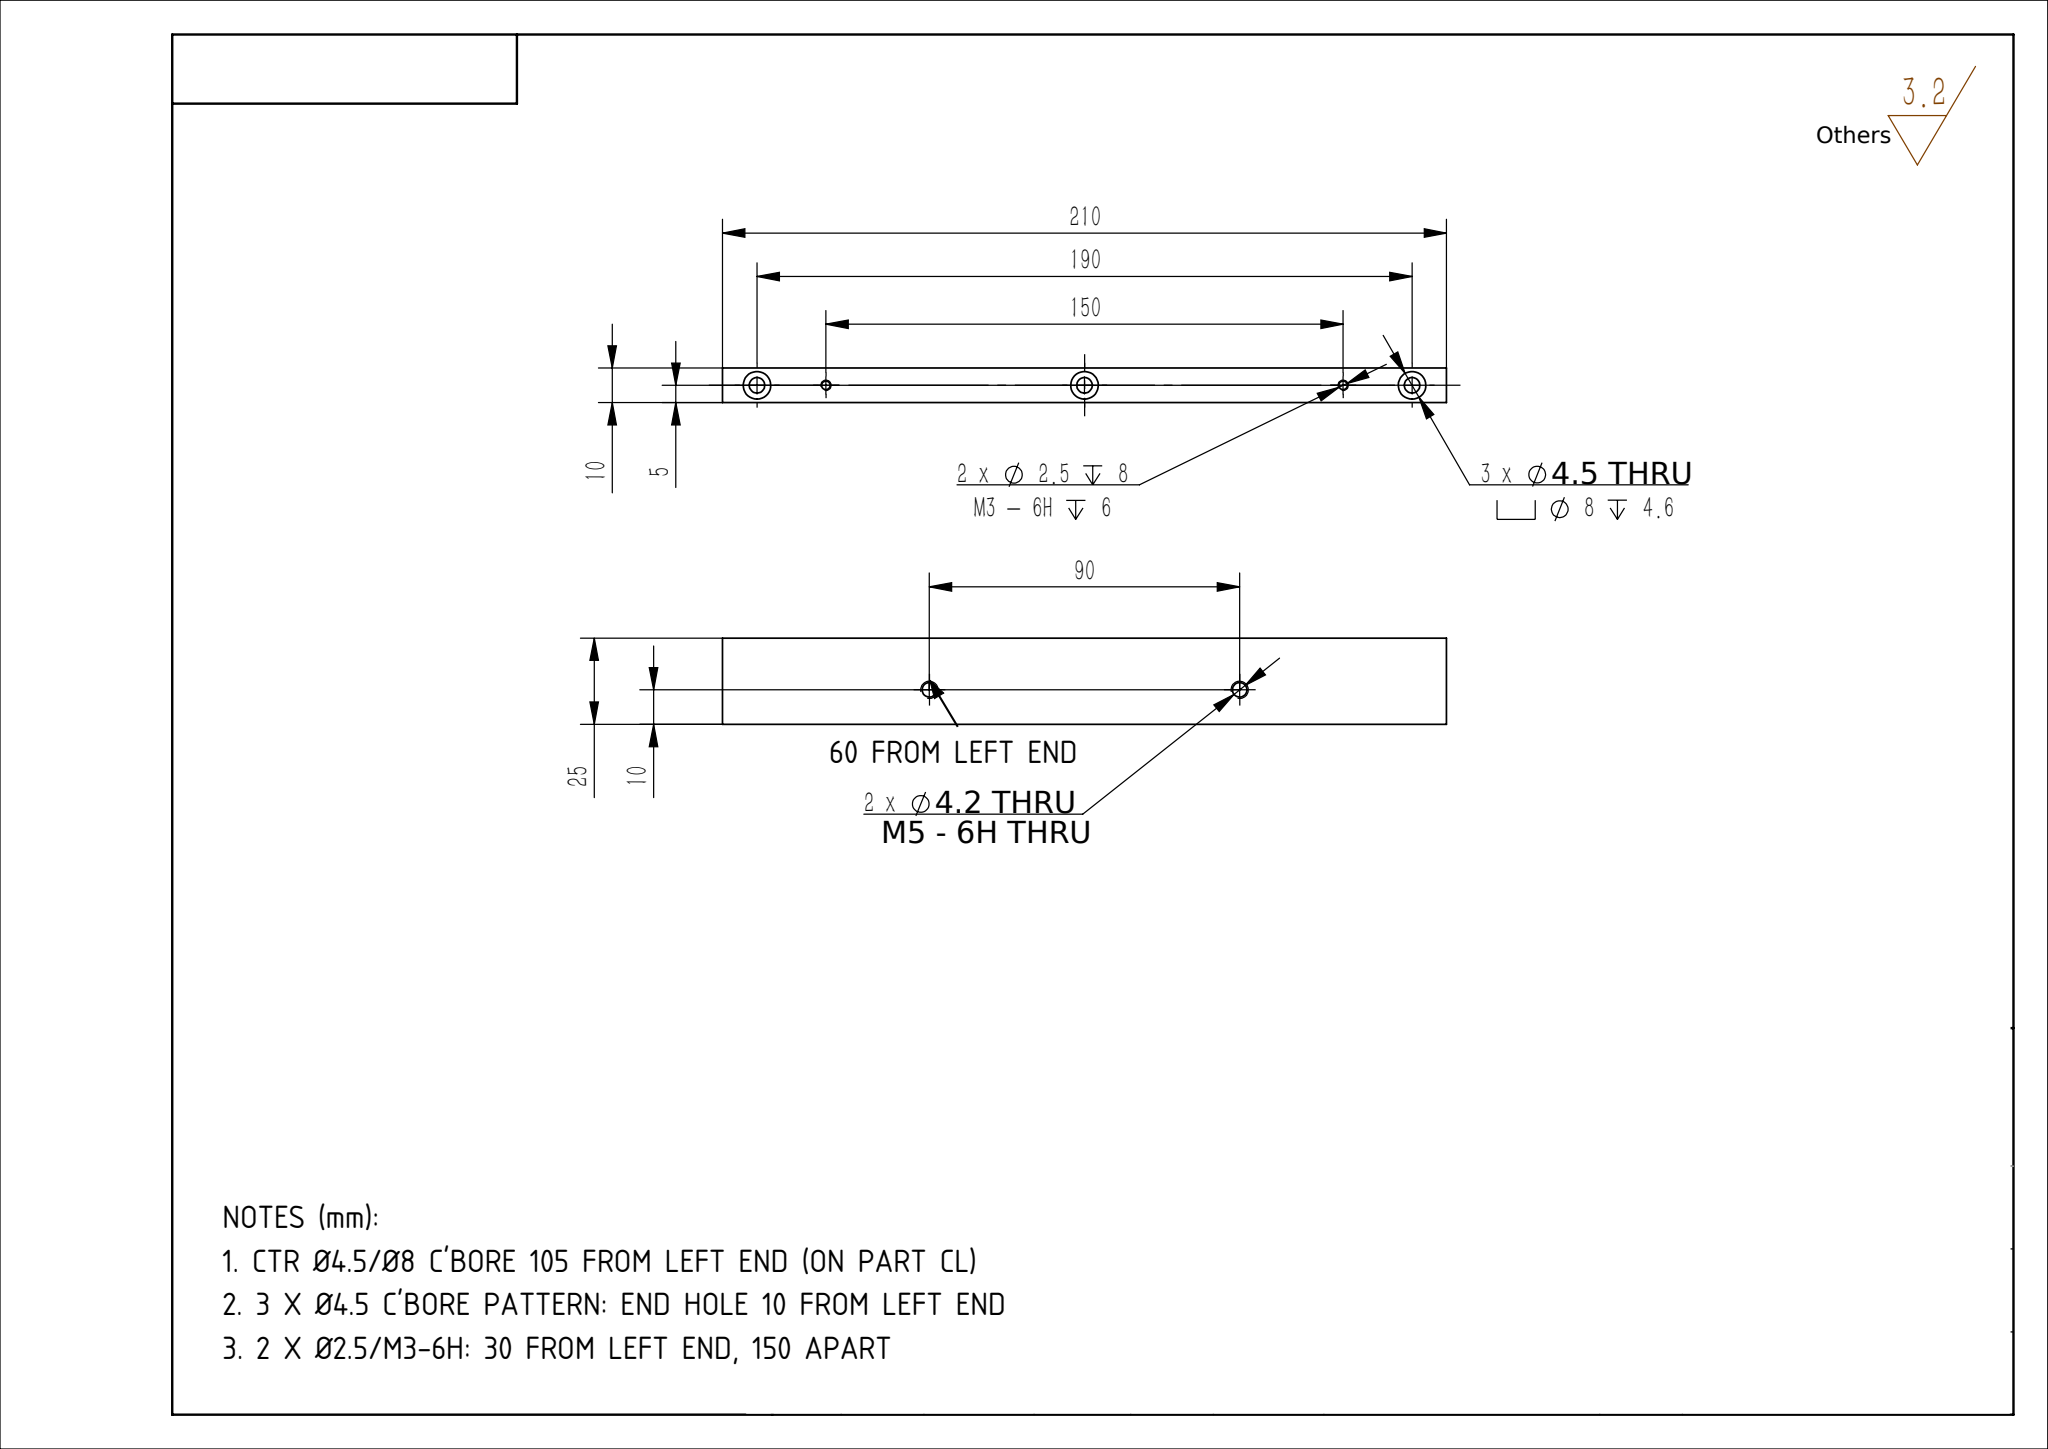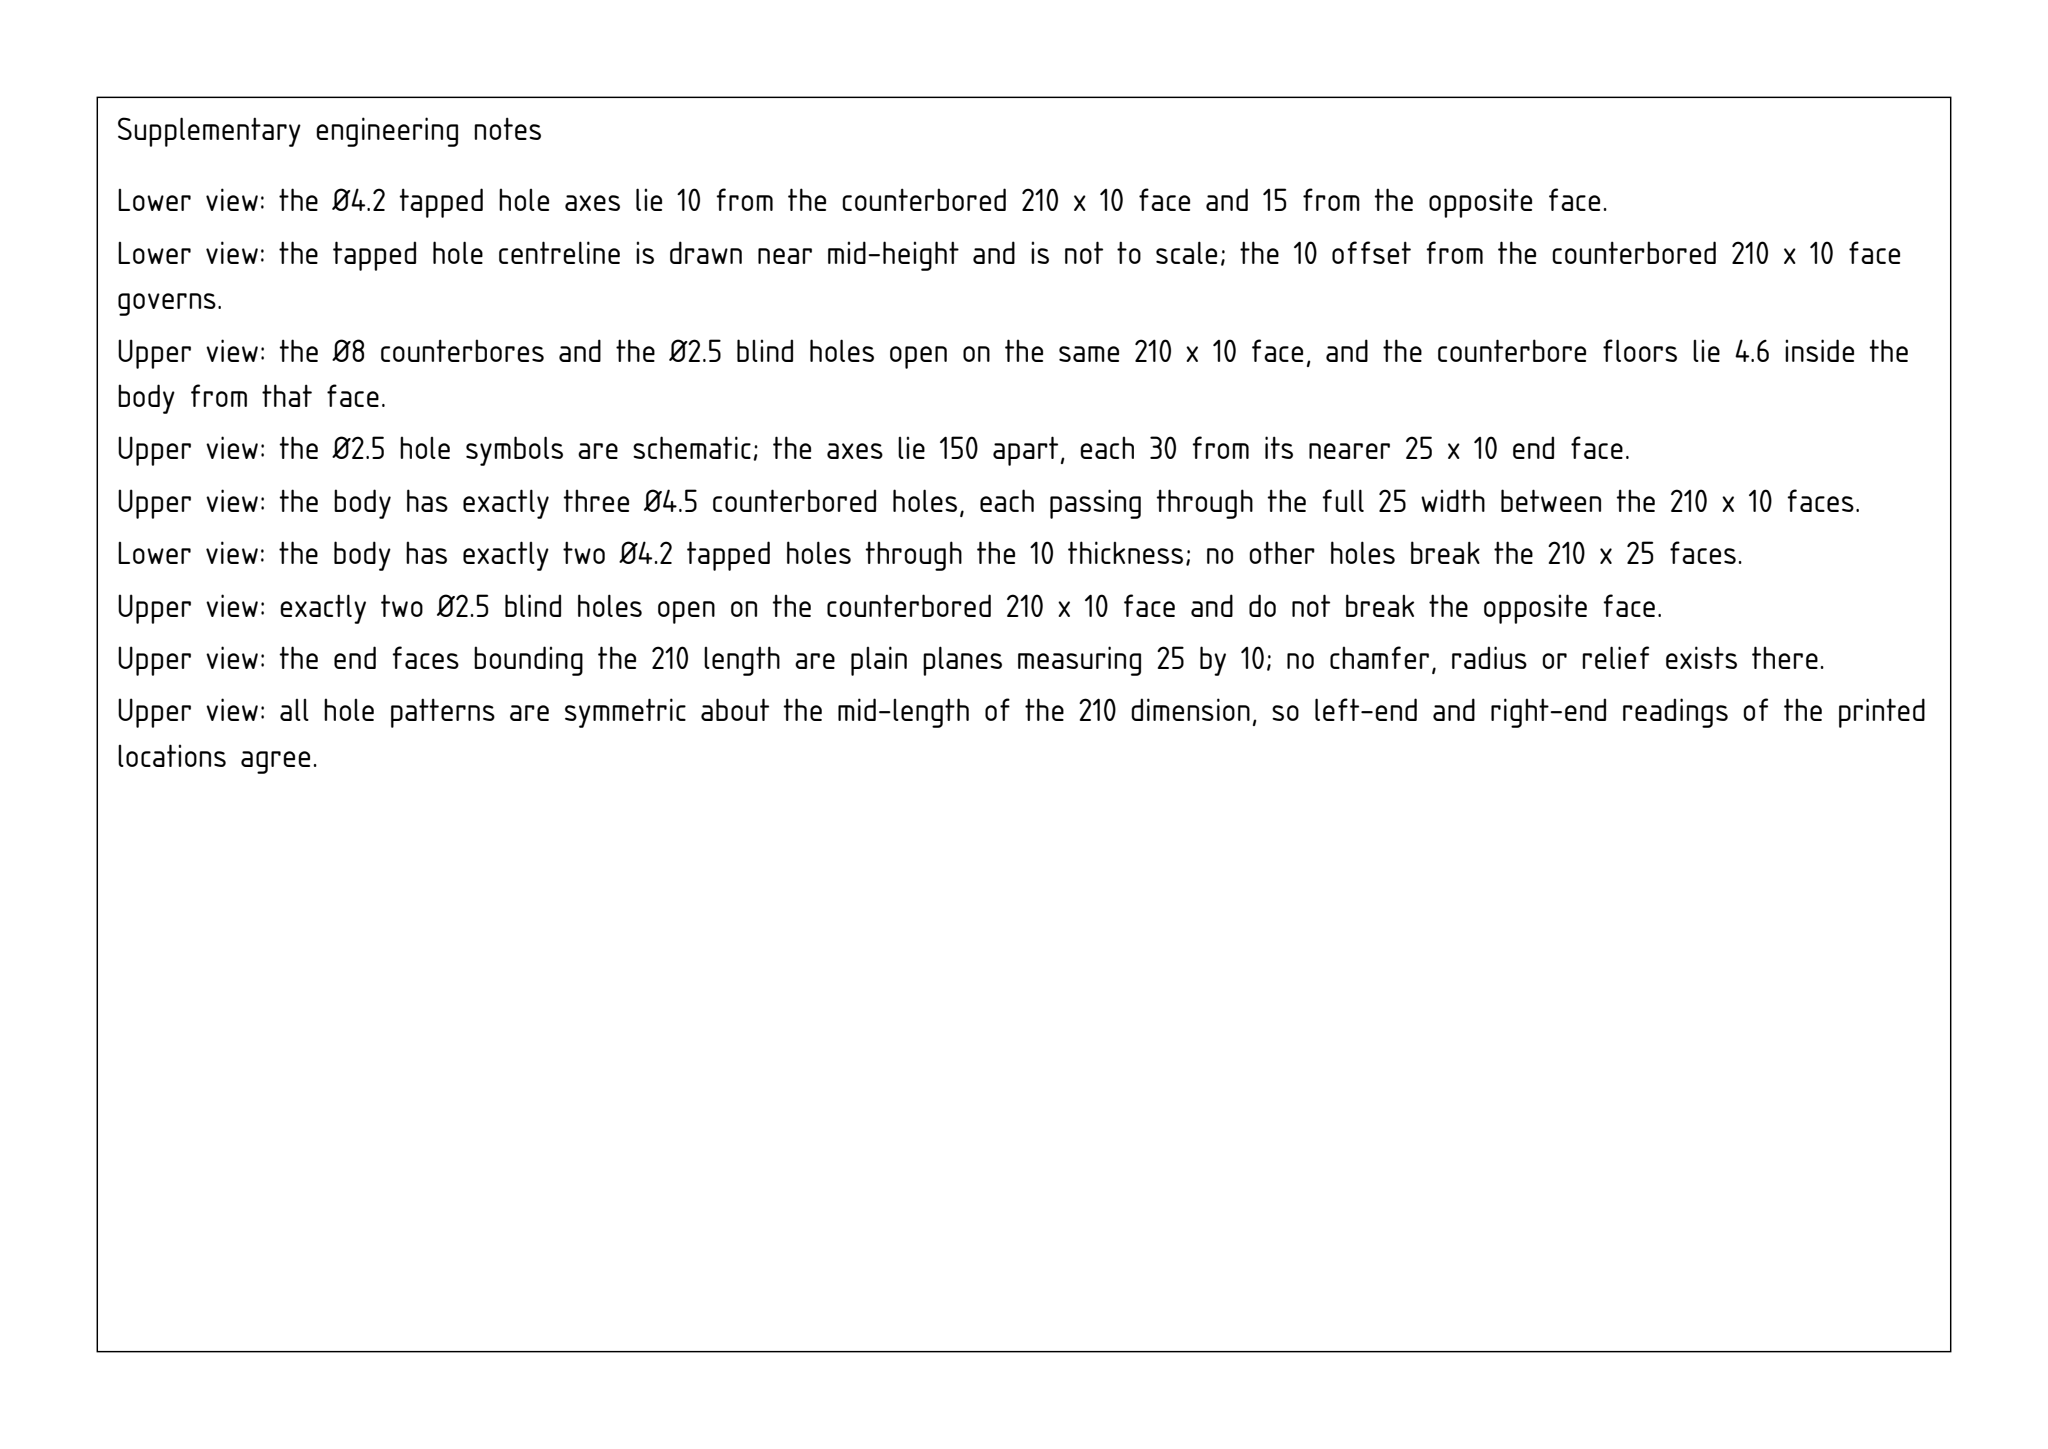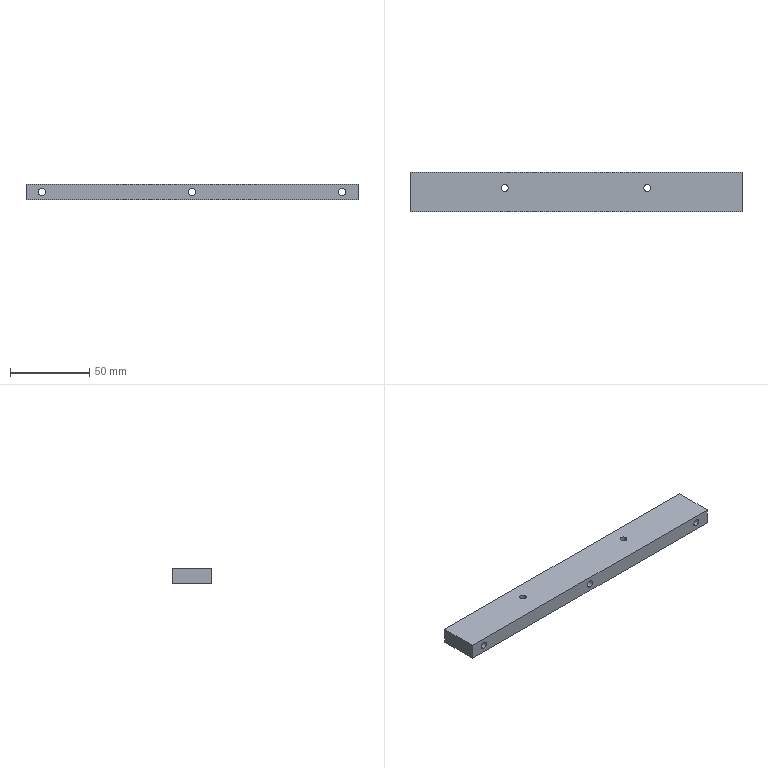Part | SolidWorks | mm | 1 solid | 33 faces | box 210 x 25 x 10 mm | volume 50475 mm3 | cylinder 20 | plane 9 | cone 4 | commonest cylinder face diameters 8 x6 4.5 x6 2.5 x4 4.2 x4
Drawing notes:
CTR Ø4.5/Ø8 C'BORE 105 FROM LEFT END (ON PART CL) | from the solid: Ø4.5/Ø8 at x=105.0; bbox x=210.0, so x=105 is midpoint
3 X Ø4.5 C'BORE PATTERN: END HOLE 10 FROM LEFT END | from the solid: Ø4.5 holes at x=10.0, 105.0, 200.0; 190 span, 10 edge dist
2 X Ø2.5/M3-6H: 30 FROM LEFT END, 150 APART | from the solid: Ø2.5 holes at x=30.0 and x=180.0
2 X Ø4.2/M5-6H: 60 FROM LEFT END, 90 APART | from the solid: Ø4.2 holes at x=60.0 and x=150.0
build123d program:
from build123d import *

# Parameters (mm, degrees)
SKETCH1_W                                         = 210
SKETCH1_H                                         = 10
BOSS_EXTRUDE1_DEPTH                               = 25
HOLE_SIZE_ACCORDING_TO_TYPE_1_HEXAGON_D           = 4.5
HOLE_SIZE_ACCORDING_TO_TYPE_1_HEXAGON_CBORE_D     = 8
HOLE_SIZE_ACCORDING_TO_TYPE_1_HEXAGON_CBORE_DEPTH = 4.6
M5_TAPPED_HOLE1_D                                 = 4.2
M3_TAPPED_HOLE1_D                                 = 2.5
M3_TAPPED_HOLE1_DEPTH                             = 8
M3_TAPPED_HOLE1_TIP                               = 0.7511


with BuildPart() as part:
    # Sketch1 → Boss-Extrude1 (new body)
    with BuildSketch(Plane(origin=(0, 0, 0), x_dir=(1, 0, 0), z_dir=(0, 1, 0))):
        Rectangle(SKETCH1_W, SKETCH1_H)
    extrude(amount=BOSS_EXTRUDE1_DEPTH)

    # Hole Size _ according to_ Type 1 Hexagon (through all)
    with Locations(Plane(origin=(0, 25, 0), x_dir=(1, 0, 0), z_dir=(0, 1, 0))):
        with Locations((-95, 0), (0, 0), (95, 0)):
            CounterBoreHole(HOLE_SIZE_ACCORDING_TO_TYPE_1_HEXAGON_D / 2, HOLE_SIZE_ACCORDING_TO_TYPE_1_HEXAGON_CBORE_D / 2, HOLE_SIZE_ACCORDING_TO_TYPE_1_HEXAGON_CBORE_DEPTH)

    # M5 Tapped Hole1 (through all)
    with Locations(Plane.XY.offset(5)):
        with Locations((-45, 15), (45, 15)):
            Hole(M5_TAPPED_HOLE1_D / 2)

    # M3 Tapped Hole1
    with Locations(Plane(origin=(0, 25, 0), x_dir=(1, 0, 0), z_dir=(0, 1, 0))):
        with Locations((-75, 0), (75, 0)):
            Hole(M3_TAPPED_HOLE1_D / 2, depth=M3_TAPPED_HOLE1_DEPTH)
            with Locations((0, 0, -(M3_TAPPED_HOLE1_DEPTH + M3_TAPPED_HOLE1_TIP / 2))):  # 118° drill point
                Cone(0, M3_TAPPED_HOLE1_D / 2, M3_TAPPED_HOLE1_TIP, mode=Mode.SUBTRACT)


solid = part.part